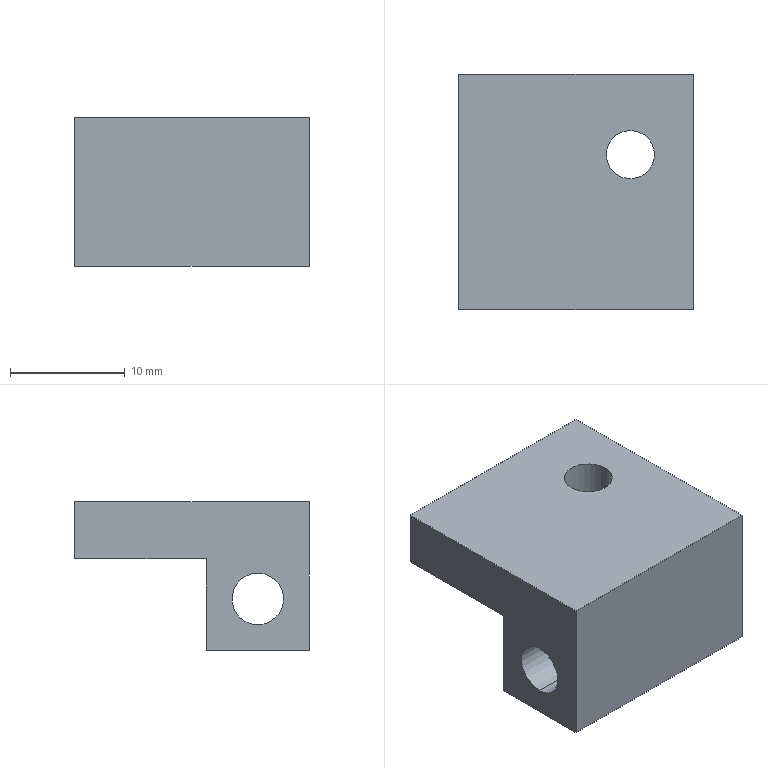Component | SolidWorks | AS-011-JG0138-1 | 1 solid | 12 faces | box 20.5 x 20.5 x 13 mm | volume 3182 mm3 | plane 8 | cylinder 4 | commonest cylinder face diameters 4.2 x2 4.5 x2
STEP:
#1=COLOUR_RGB('',0.7922,0.8196,0.9333);
#2=FILL_AREA_STYLE_COLOUR('',#1);
#3=FILL_AREA_STYLE('',(#2));
#4=SURFACE_STYLE_FILL_AREA(#3);
#5=SURFACE_SIDE_STYLE('',(#4));
#6=SURFACE_STYLE_USAGE(.BOTH.,#5);
#7=PRESENTATION_STYLE_ASSIGNMENT((#6));
#8=CARTESIAN_POINT('',(-0.6732,-1.102,0.3346));
#9=VERTEX_POINT('',#8);
#10=CARTESIAN_POINT('',(-0.5079,-1.102,0.3346));
#11=VERTEX_POINT('',#10);
#12=CARTESIAN_POINT('',(-0.5906,-1.102,0.3346));
#13=DIRECTION('',(0.,0.,1.));
#14=DIRECTION('',(1.,0.,0.));
#15=AXIS2_PLACEMENT_3D('',#12,#13,#14);
#16=CIRCLE('',#15,0.08268);
#17=EDGE_CURVE('',#9,#11,#16,.T.);
#18=ORIENTED_EDGE('',*,*,#17,.F.);
#19=CARTESIAN_POINT('',(-0.6732,-1.102,0.5315));
#20=VERTEX_POINT('',#19);
#21=CARTESIAN_POINT('',(-0.6732,-1.102,0.5315));
#22=DIRECTION('',(-0.,0.,1.));
#23=VECTOR('',#22,39.37);
#24=LINE('',#21,#23);
#25=EDGE_CURVE('',#9,#20,#24,.T.);
#26=ORIENTED_EDGE('',*,*,#25,.T.);
#27=CARTESIAN_POINT('',(-0.5079,-1.102,0.5315));
#28=VERTEX_POINT('',#27);
#29=CARTESIAN_POINT('',(-0.5906,-1.102,0.5315));
#30=DIRECTION('',(-0.,0.,1.));
#31=DIRECTION('',(1.,0.,0.));
#32=AXIS2_PLACEMENT_3D('',#29,#30,#31);
#33=CIRCLE('',#32,0.08268);
#34=EDGE_CURVE('',#20,#28,#33,.T.);
#35=ORIENTED_EDGE('',*,*,#34,.T.);
#36=CARTESIAN_POINT('',(-0.5079,-1.102,0.5315));
#37=DIRECTION('',(-0.,0.,1.));
#38=VECTOR('',#37,39.37);
#39=LINE('',#36,#38);
#40=EDGE_CURVE('',#11,#28,#39,.T.);
#41=ORIENTED_EDGE('',*,*,#40,.F.);
#42=EDGE_LOOP('',(#18,#26,#35,#41));
#43=FACE_OUTER_BOUND('',#42,.T.);
#44=CARTESIAN_POINT('',(-0.5906,-1.102,0.5315));
#45=DIRECTION('',(-0.,0.,1.));
#46=DIRECTION('',(1.,0.,0.));
#47=AXIS2_PLACEMENT_3D('',#44,#45,#46);
#48=CYLINDRICAL_SURFACE('',#47,0.08268);
#49=ADVANCED_FACE('',(#43),#48,.F.);
#50=CARTESIAN_POINT('',(-1.181,-1.457,0.1083));
#51=VERTEX_POINT('',#50);
#52=CARTESIAN_POINT('',(-1.181,-1.457,0.2854));
#53=VERTEX_POINT('',#52);
#54=CARTESIAN_POINT('',(-1.181,-1.457,0.1969));
#55=DIRECTION('',(-1.,0.,0.));
#56=DIRECTION('',(0.,0.,1.));
#57=AXIS2_PLACEMENT_3D('',#54,#55,#56);
#58=CIRCLE('',#57,0.08858);
#59=EDGE_CURVE('',#51,#53,#58,.T.);
#60=ORIENTED_EDGE('',*,*,#59,.T.);
#61=CARTESIAN_POINT('',(-0.374,-1.457,0.2854));
#62=VERTEX_POINT('',#61);
#63=CARTESIAN_POINT('',(-1.28,-1.457,0.2854));
#64=DIRECTION('',(1.,0.,0.));
#65=VECTOR('',#64,39.37);
#66=LINE('',#63,#65);
#67=EDGE_CURVE('',#53,#62,#66,.T.);
#68=ORIENTED_EDGE('',*,*,#67,.T.);
#69=CARTESIAN_POINT('',(-0.374,-1.457,0.1083));
#70=VERTEX_POINT('',#69);
#71=CARTESIAN_POINT('',(-0.374,-1.457,0.1969));
#72=DIRECTION('',(1.,0.,0.));
#73=DIRECTION('',(0.,0.,-1.));
#74=AXIS2_PLACEMENT_3D('',#71,#72,#73);
#75=CIRCLE('',#74,0.08858);
#76=EDGE_CURVE('',#62,#70,#75,.T.);
#77=ORIENTED_EDGE('',*,*,#76,.T.);
#78=CARTESIAN_POINT('',(-1.28,-1.457,0.1083));
#79=DIRECTION('',(1.,0.,0.));
#80=VECTOR('',#79,39.37);
#81=LINE('',#78,#80);
#82=EDGE_CURVE('',#51,#70,#81,.T.);
#83=ORIENTED_EDGE('',*,*,#82,.F.);
#84=EDGE_LOOP('',(#60,#68,#77,#83));
#85=FACE_OUTER_BOUND('',#84,.T.);
#86=CARTESIAN_POINT('',(-1.28,-1.457,0.1969));
#87=DIRECTION('',(1.,0.,0.));
#88=DIRECTION('',(0.,0.,-1.));
#89=AXIS2_PLACEMENT_3D('',#86,#87,#88);
#90=CYLINDRICAL_SURFACE('',#89,0.08858);
#91=ADVANCED_FACE('',(#85),#90,.F.);
#92=ORIENTED_EDGE('',*,*,#59,.F.);
#93=CARTESIAN_POINT('',(-1.181,-1.457,0.1969));
#94=DIRECTION('',(-1.,0.,0.));
#95=DIRECTION('',(0.,0.,1.));
#96=AXIS2_PLACEMENT_3D('',#93,#94,#95);
#97=CIRCLE('',#96,0.08858);
#98=EDGE_CURVE('',#53,#51,#97,.T.);
#99=ORIENTED_EDGE('',*,*,#98,.F.);
#100=EDGE_LOOP('',(#92,#99));
#101=FACE_BOUND('',#100,.T.);
#102=CARTESIAN_POINT('',(-1.181,-1.634,0.01969));
#103=VERTEX_POINT('',#102);
#104=CARTESIAN_POINT('',(-1.181,-1.634,0.5315));
#105=VERTEX_POINT('',#104);
#106=CARTESIAN_POINT('',(-1.181,-1.634,0.01969));
#107=DIRECTION('',(0.,0.,1.));
#108=VECTOR('',#107,39.37);
#109=LINE('',#106,#108);
#110=EDGE_CURVE('',#103,#105,#109,.T.);
#111=ORIENTED_EDGE('',*,*,#110,.T.);
#112=CARTESIAN_POINT('',(-1.181,-0.8268,0.5315));
#113=VERTEX_POINT('',#112);
#114=CARTESIAN_POINT('',(-1.181,-0.8268,0.5315));
#115=DIRECTION('',(0.,-1.,0.));
#116=VECTOR('',#115,39.37);
#117=LINE('',#114,#116);
#118=EDGE_CURVE('',#113,#105,#117,.T.);
#119=ORIENTED_EDGE('',*,*,#118,.F.);
#120=CARTESIAN_POINT('',(-1.181,-0.8268,0.3346));
#121=VERTEX_POINT('',#120);
#122=CARTESIAN_POINT('',(-1.181,-0.8268,0.01969));
#123=DIRECTION('',(0.,0.,1.));
#124=VECTOR('',#123,39.37);
#125=LINE('',#122,#124);
#126=EDGE_CURVE('',#121,#113,#125,.T.);
#127=ORIENTED_EDGE('',*,*,#126,.F.);
#128=CARTESIAN_POINT('',(-1.181,-1.28,0.3346));
#129=VERTEX_POINT('',#128);
#130=CARTESIAN_POINT('',(-1.181,-0.8268,0.3346));
#131=DIRECTION('',(0.,1.,0.));
#132=VECTOR('',#131,39.37);
#133=LINE('',#130,#132);
#134=EDGE_CURVE('',#129,#121,#133,.T.);
#135=ORIENTED_EDGE('',*,*,#134,.F.);
#136=CARTESIAN_POINT('',(-1.181,-1.28,0.01969));
#137=VERTEX_POINT('',#136);
#138=CARTESIAN_POINT('',(-1.181,-1.28,0.01969));
#139=DIRECTION('',(0.,0.,1.));
#140=VECTOR('',#139,39.37);
#141=LINE('',#138,#140);
#142=EDGE_CURVE('',#137,#129,#141,.T.);
#143=ORIENTED_EDGE('',*,*,#142,.F.);
#144=CARTESIAN_POINT('',(-1.181,-0.8268,0.01969));
#145=DIRECTION('',(0.,-1.,0.));
#146=VECTOR('',#145,39.37);
#147=LINE('',#144,#146);
#148=EDGE_CURVE('',#137,#103,#147,.T.);
#149=ORIENTED_EDGE('',*,*,#148,.T.);
#150=EDGE_LOOP('',(#111,#119,#127,#135,#143,#149));
#151=FACE_OUTER_BOUND('',#150,.T.);
#152=CARTESIAN_POINT('',(-1.181,-0.8268,0.01969));
#153=DIRECTION('',(-1.,0.,0.));
#154=DIRECTION('',(0.,0.,1.));
#155=AXIS2_PLACEMENT_3D('',#152,#153,#154);
#156=PLANE('',#155);
#157=ADVANCED_FACE('',(#101,#151),#156,.T.);
#158=ORIENTED_EDGE('',*,*,#126,.T.);
#159=CARTESIAN_POINT('',(-0.374,-0.8268,0.5315));
#160=VERTEX_POINT('',#159);
#161=CARTESIAN_POINT('',(-0.374,-0.8268,0.5315));
#162=DIRECTION('',(-1.,0.,0.));
#163=VECTOR('',#162,39.37);
#164=LINE('',#161,#163);
#165=EDGE_CURVE('',#160,#113,#164,.T.);
#166=ORIENTED_EDGE('',*,*,#165,.F.);
#167=CARTESIAN_POINT('',(-0.374,-0.8268,0.3346));
#168=VERTEX_POINT('',#167);
#169=CARTESIAN_POINT('',(-0.374,-0.8268,0.01969));
#170=DIRECTION('',(0.,0.,1.));
#171=VECTOR('',#170,39.37);
#172=LINE('',#169,#171);
#173=EDGE_CURVE('',#168,#160,#172,.T.);
#174=ORIENTED_EDGE('',*,*,#173,.F.);
#175=CARTESIAN_POINT('',(-1.28,-0.8268,0.3346));
#176=DIRECTION('',(1.,0.,0.));
#177=VECTOR('',#176,39.37);
#178=LINE('',#175,#177);
#179=EDGE_CURVE('',#121,#168,#178,.T.);
#180=ORIENTED_EDGE('',*,*,#179,.F.);
#181=EDGE_LOOP('',(#158,#166,#174,#180));
#182=FACE_OUTER_BOUND('',#181,.T.);
#183=CARTESIAN_POINT('',(-0.374,-0.8268,0.01969));
#184=DIRECTION('',(0.,1.,0.));
#185=DIRECTION('',(0.,0.,1.));
#186=AXIS2_PLACEMENT_3D('',#183,#184,#185);
#187=PLANE('',#186);
#188=ADVANCED_FACE('',(#182),#187,.T.);
#189=CARTESIAN_POINT('',(-0.374,-1.457,0.1969));
#190=DIRECTION('',(1.,0.,0.));
#191=DIRECTION('',(0.,0.,-1.));
#192=AXIS2_PLACEMENT_3D('',#189,#190,#191);
#193=CIRCLE('',#192,0.08858);
#194=EDGE_CURVE('',#70,#62,#193,.T.);
#195=ORIENTED_EDGE('',*,*,#194,.F.);
#196=ORIENTED_EDGE('',*,*,#76,.F.);
#197=EDGE_LOOP('',(#195,#196));
#198=FACE_BOUND('',#197,.T.);
#199=ORIENTED_EDGE('',*,*,#173,.T.);
#200=CARTESIAN_POINT('',(-0.374,-1.634,0.5315));
#201=VERTEX_POINT('',#200);
#202=CARTESIAN_POINT('',(-0.374,-1.634,0.5315));
#203=DIRECTION('',(0.,1.,0.));
#204=VECTOR('',#203,39.37);
#205=LINE('',#202,#204);
#206=EDGE_CURVE('',#201,#160,#205,.T.);
#207=ORIENTED_EDGE('',*,*,#206,.F.);
#208=CARTESIAN_POINT('',(-0.374,-1.634,0.01969));
#209=VERTEX_POINT('',#208);
#210=CARTESIAN_POINT('',(-0.374,-1.634,0.01969));
#211=DIRECTION('',(0.,0.,1.));
#212=VECTOR('',#211,39.37);
#213=LINE('',#210,#212);
#214=EDGE_CURVE('',#209,#201,#213,.T.);
#215=ORIENTED_EDGE('',*,*,#214,.F.);
#216=CARTESIAN_POINT('',(-0.374,-1.28,0.01969));
#217=VERTEX_POINT('',#216);
#218=CARTESIAN_POINT('',(-0.374,-0.8268,0.01969));
#219=DIRECTION('',(0.,1.,0.));
#220=VECTOR('',#219,39.37);
#221=LINE('',#218,#220);
#222=EDGE_CURVE('',#209,#217,#221,.T.);
#223=ORIENTED_EDGE('',*,*,#222,.T.);
#224=CARTESIAN_POINT('',(-0.374,-1.28,0.3346));
#225=VERTEX_POINT('',#224);
#226=CARTESIAN_POINT('',(-0.374,-1.28,0.9252));
#227=DIRECTION('',(0.,0.,-1.));
#228=VECTOR('',#227,39.37);
#229=LINE('',#226,#228);
#230=EDGE_CURVE('',#225,#217,#229,.T.);
#231=ORIENTED_EDGE('',*,*,#230,.F.);
#232=CARTESIAN_POINT('',(-0.374,-0.8268,0.3346));
#233=DIRECTION('',(0.,-1.,0.));
#234=VECTOR('',#233,39.37);
#235=LINE('',#232,#234);
#236=EDGE_CURVE('',#168,#225,#235,.T.);
#237=ORIENTED_EDGE('',*,*,#236,.F.);
#238=EDGE_LOOP('',(#199,#207,#215,#223,#231,#237));
#239=FACE_OUTER_BOUND('',#238,.T.);
#240=CARTESIAN_POINT('',(-0.374,-0.8268,0.01969));
#241=DIRECTION('',(1.,0.,0.));
#242=DIRECTION('',(0.,0.,-1.));
#243=AXIS2_PLACEMENT_3D('',#240,#241,#242);
#244=PLANE('',#243);
#245=ADVANCED_FACE('',(#198,#239),#244,.T.);
#246=CARTESIAN_POINT('',(-1.181,-1.634,0.5315));
#247=DIRECTION('',(1.,0.,0.));
#248=VECTOR('',#247,39.37);
#249=LINE('',#246,#248);
#250=EDGE_CURVE('',#105,#201,#249,.T.);
#251=ORIENTED_EDGE('',*,*,#250,.F.);
#252=ORIENTED_EDGE('',*,*,#110,.F.);
#253=CARTESIAN_POINT('',(-0.374,-1.634,0.01969));
#254=DIRECTION('',(-1.,0.,0.));
#255=VECTOR('',#254,39.37);
#256=LINE('',#253,#255);
#257=EDGE_CURVE('',#209,#103,#256,.T.);
#258=ORIENTED_EDGE('',*,*,#257,.F.);
#259=ORIENTED_EDGE('',*,*,#214,.T.);
#260=EDGE_LOOP('',(#251,#252,#258,#259));
#261=FACE_OUTER_BOUND('',#260,.T.);
#262=CARTESIAN_POINT('',(-0.374,-1.634,0.01969));
#263=DIRECTION('',(0.,1.,0.));
#264=DIRECTION('',(0.,0.,1.));
#265=AXIS2_PLACEMENT_3D('',#262,#263,#264);
#266=PLANE('',#265);
#267=ADVANCED_FACE('',(#261),#266,.F.);
#268=ORIENTED_EDGE('',*,*,#148,.F.);
#269=CARTESIAN_POINT('',(-0.374,-1.28,0.01969));
#270=DIRECTION('',(1.,0.,0.));
#271=VECTOR('',#270,39.37);
#272=LINE('',#269,#271);
#273=EDGE_CURVE('',#137,#217,#272,.T.);
#274=ORIENTED_EDGE('',*,*,#273,.T.);
#275=ORIENTED_EDGE('',*,*,#222,.F.);
#276=ORIENTED_EDGE('',*,*,#257,.T.);
#277=EDGE_LOOP('',(#268,#274,#275,#276));
#278=FACE_OUTER_BOUND('',#277,.T.);
#279=CARTESIAN_POINT('',(-0.374,-0.8268,0.01969));
#280=DIRECTION('',(0.,0.,1.));
#281=DIRECTION('',(1.,0.,0.));
#282=AXIS2_PLACEMENT_3D('',#279,#280,#281);
#283=PLANE('',#282);
#284=ADVANCED_FACE('',(#278),#283,.F.);
#285=ORIENTED_EDGE('',*,*,#142,.T.);
#286=CARTESIAN_POINT('',(-1.28,-1.28,0.3346));
#287=DIRECTION('',(1.,0.,0.));
#288=VECTOR('',#287,39.37);
#289=LINE('',#286,#288);
#290=EDGE_CURVE('',#129,#225,#289,.T.);
#291=ORIENTED_EDGE('',*,*,#290,.T.);
#292=ORIENTED_EDGE('',*,*,#230,.T.);
#293=ORIENTED_EDGE('',*,*,#273,.F.);
#294=EDGE_LOOP('',(#285,#291,#292,#293));
#295=FACE_OUTER_BOUND('',#294,.T.);
#296=CARTESIAN_POINT('',(-1.28,-1.28,0.9252));
#297=DIRECTION('',(0.,-1.,0.));
#298=DIRECTION('',(0.,0.,-1.));
#299=AXIS2_PLACEMENT_3D('',#296,#297,#298);
#300=PLANE('',#299);
#301=ADVANCED_FACE('',(#295),#300,.F.);
#302=CARTESIAN_POINT('',(-0.5906,-1.102,0.3346));
#303=DIRECTION('',(0.,0.,1.));
#304=DIRECTION('',(1.,0.,0.));
#305=AXIS2_PLACEMENT_3D('',#302,#303,#304);
#306=CIRCLE('',#305,0.08268);
#307=EDGE_CURVE('',#11,#9,#306,.T.);
#308=ORIENTED_EDGE('',*,*,#307,.T.);
#309=ORIENTED_EDGE('',*,*,#17,.T.);
#310=EDGE_LOOP('',(#308,#309));
#311=FACE_BOUND('',#310,.T.);
#312=ORIENTED_EDGE('',*,*,#290,.F.);
#313=ORIENTED_EDGE('',*,*,#134,.T.);
#314=ORIENTED_EDGE('',*,*,#179,.T.);
#315=ORIENTED_EDGE('',*,*,#236,.T.);
#316=EDGE_LOOP('',(#312,#313,#314,#315));
#317=FACE_OUTER_BOUND('',#316,.T.);
#318=CARTESIAN_POINT('',(-1.28,-0.8268,0.3346));
#319=DIRECTION('',(0.,0.,1.));
#320=DIRECTION('',(1.,0.,0.));
#321=AXIS2_PLACEMENT_3D('',#318,#319,#320);
#322=PLANE('',#321);
#323=ADVANCED_FACE('',(#311,#317),#322,.F.);
#324=ORIENTED_EDGE('',*,*,#67,.F.);
#325=ORIENTED_EDGE('',*,*,#98,.T.);
#326=ORIENTED_EDGE('',*,*,#82,.T.);
#327=ORIENTED_EDGE('',*,*,#194,.T.);
#328=EDGE_LOOP('',(#324,#325,#326,#327));
#329=FACE_OUTER_BOUND('',#328,.T.);
#330=CARTESIAN_POINT('',(-1.28,-1.457,0.1969));
#331=DIRECTION('',(1.,0.,0.));
#332=DIRECTION('',(0.,0.,-1.));
#333=AXIS2_PLACEMENT_3D('',#330,#331,#332);
#334=CYLINDRICAL_SURFACE('',#333,0.08858);
#335=ADVANCED_FACE('',(#329),#334,.F.);
#336=CARTESIAN_POINT('',(-0.5906,-1.102,0.5315));
#337=DIRECTION('',(-0.,0.,1.));
#338=DIRECTION('',(1.,0.,0.));
#339=AXIS2_PLACEMENT_3D('',#336,#337,#338);
#340=CIRCLE('',#339,0.08268);
#341=EDGE_CURVE('',#28,#20,#340,.T.);
#342=ORIENTED_EDGE('',*,*,#341,.F.);
#343=ORIENTED_EDGE('',*,*,#34,.F.);
#344=EDGE_LOOP('',(#342,#343));
#345=FACE_BOUND('',#344,.T.);
#346=ORIENTED_EDGE('',*,*,#250,.T.);
#347=ORIENTED_EDGE('',*,*,#206,.T.);
#348=ORIENTED_EDGE('',*,*,#165,.T.);
#349=ORIENTED_EDGE('',*,*,#118,.T.);
#350=EDGE_LOOP('',(#346,#347,#348,#349));
#351=FACE_OUTER_BOUND('',#350,.T.);
#352=CARTESIAN_POINT('',(-0.374,-0.8268,0.5315));
#353=DIRECTION('',(0.,0.,1.));
#354=DIRECTION('',(1.,0.,0.));
#355=AXIS2_PLACEMENT_3D('',#352,#353,#354);
#356=PLANE('',#355);
#357=ADVANCED_FACE('',(#345,#351),#356,.T.);
#358=ORIENTED_EDGE('',*,*,#25,.F.);
#359=ORIENTED_EDGE('',*,*,#307,.F.);
#360=ORIENTED_EDGE('',*,*,#40,.T.);
#361=ORIENTED_EDGE('',*,*,#341,.T.);
#362=EDGE_LOOP('',(#358,#359,#360,#361));
#363=FACE_OUTER_BOUND('',#362,.T.);
#364=CARTESIAN_POINT('',(-0.5906,-1.102,0.5315));
#365=DIRECTION('',(-0.,0.,1.));
#366=DIRECTION('',(1.,0.,0.));
#367=AXIS2_PLACEMENT_3D('',#364,#365,#366);
#368=CYLINDRICAL_SURFACE('',#367,0.08268);
#369=ADVANCED_FACE('',(#363),#368,.F.);
#370=CLOSED_SHELL('',(#49,#91,#157,#188,#245,#267,#284,#301,#323,#335,#357,#369));
#371=MANIFOLD_SOLID_BREP('',#370);
#372=STYLED_ITEM('',(#7),#371);
#373=PRESENTATION_LAYER_ASSIGNMENT('','',(#372));
#374=CARTESIAN_POINT('',(0.,0.,0.));
#375=DIRECTION('',(0.,0.,1.));
#376=DIRECTION('',(1.,0.,0.));
#377=AXIS2_PLACEMENT_3D('',#374,#375,#376);
#378=(LENGTH_UNIT()NAMED_UNIT(*)SI_UNIT($,.METRE.));
#379=LENGTH_MEASURE_WITH_UNIT(LENGTH_MEASURE(0.0254),#378);
#380=DIMENSIONAL_EXPONENTS(1.,0.,0.,0.,0.,0.,0.);
#381=(CONVERSION_BASED_UNIT('',#379)LENGTH_UNIT()NAMED_UNIT(#380));
#382=UNCERTAINTY_MEASURE_WITH_UNIT(LENGTH_MEASURE(0.00001),#381,'','');
#383=(NAMED_UNIT(*)PLANE_ANGLE_UNIT()SI_UNIT($,.RADIAN.));
#384=(NAMED_UNIT(*)SI_UNIT($,.STERADIAN.)SOLID_ANGLE_UNIT());
#385=(GEOMETRIC_REPRESENTATION_CONTEXT(3)GLOBAL_UNCERTAINTY_ASSIGNED_CONTEXT((#382))GLOBAL_UNIT_ASSIGNED_CONTEXT((#381,#383,#384))REPRESENTATION_CONTEXT('',''));
#386=ADVANCED_BREP_SHAPE_REPRESENTATION('',(#371,#377),#385);
#387=(LENGTH_UNIT()NAMED_UNIT(*)SI_UNIT($,.METRE.));
#388=LENGTH_MEASURE_WITH_UNIT(LENGTH_MEASURE(0.0254),#387);
#389=DIMENSIONAL_EXPONENTS(1.,0.,0.,0.,0.,0.,0.);
#390=(CONVERSION_BASED_UNIT('',#388)LENGTH_UNIT()NAMED_UNIT(#389));
#391=UNCERTAINTY_MEASURE_WITH_UNIT(LENGTH_MEASURE(0.00001),#390,'','');
#392=(NAMED_UNIT(*)PLANE_ANGLE_UNIT()SI_UNIT($,.RADIAN.));
#393=(NAMED_UNIT(*)SI_UNIT($,.STERADIAN.)SOLID_ANGLE_UNIT());
#394=(GEOMETRIC_REPRESENTATION_CONTEXT(3)GLOBAL_UNCERTAINTY_ASSIGNED_CONTEXT((#391))GLOBAL_UNIT_ASSIGNED_CONTEXT((#390,#392,#393))REPRESENTATION_CONTEXT('',''));
#395=MECHANICAL_DESIGN_GEOMETRIC_PRESENTATION_REPRESENTATION('',(#372),#394);